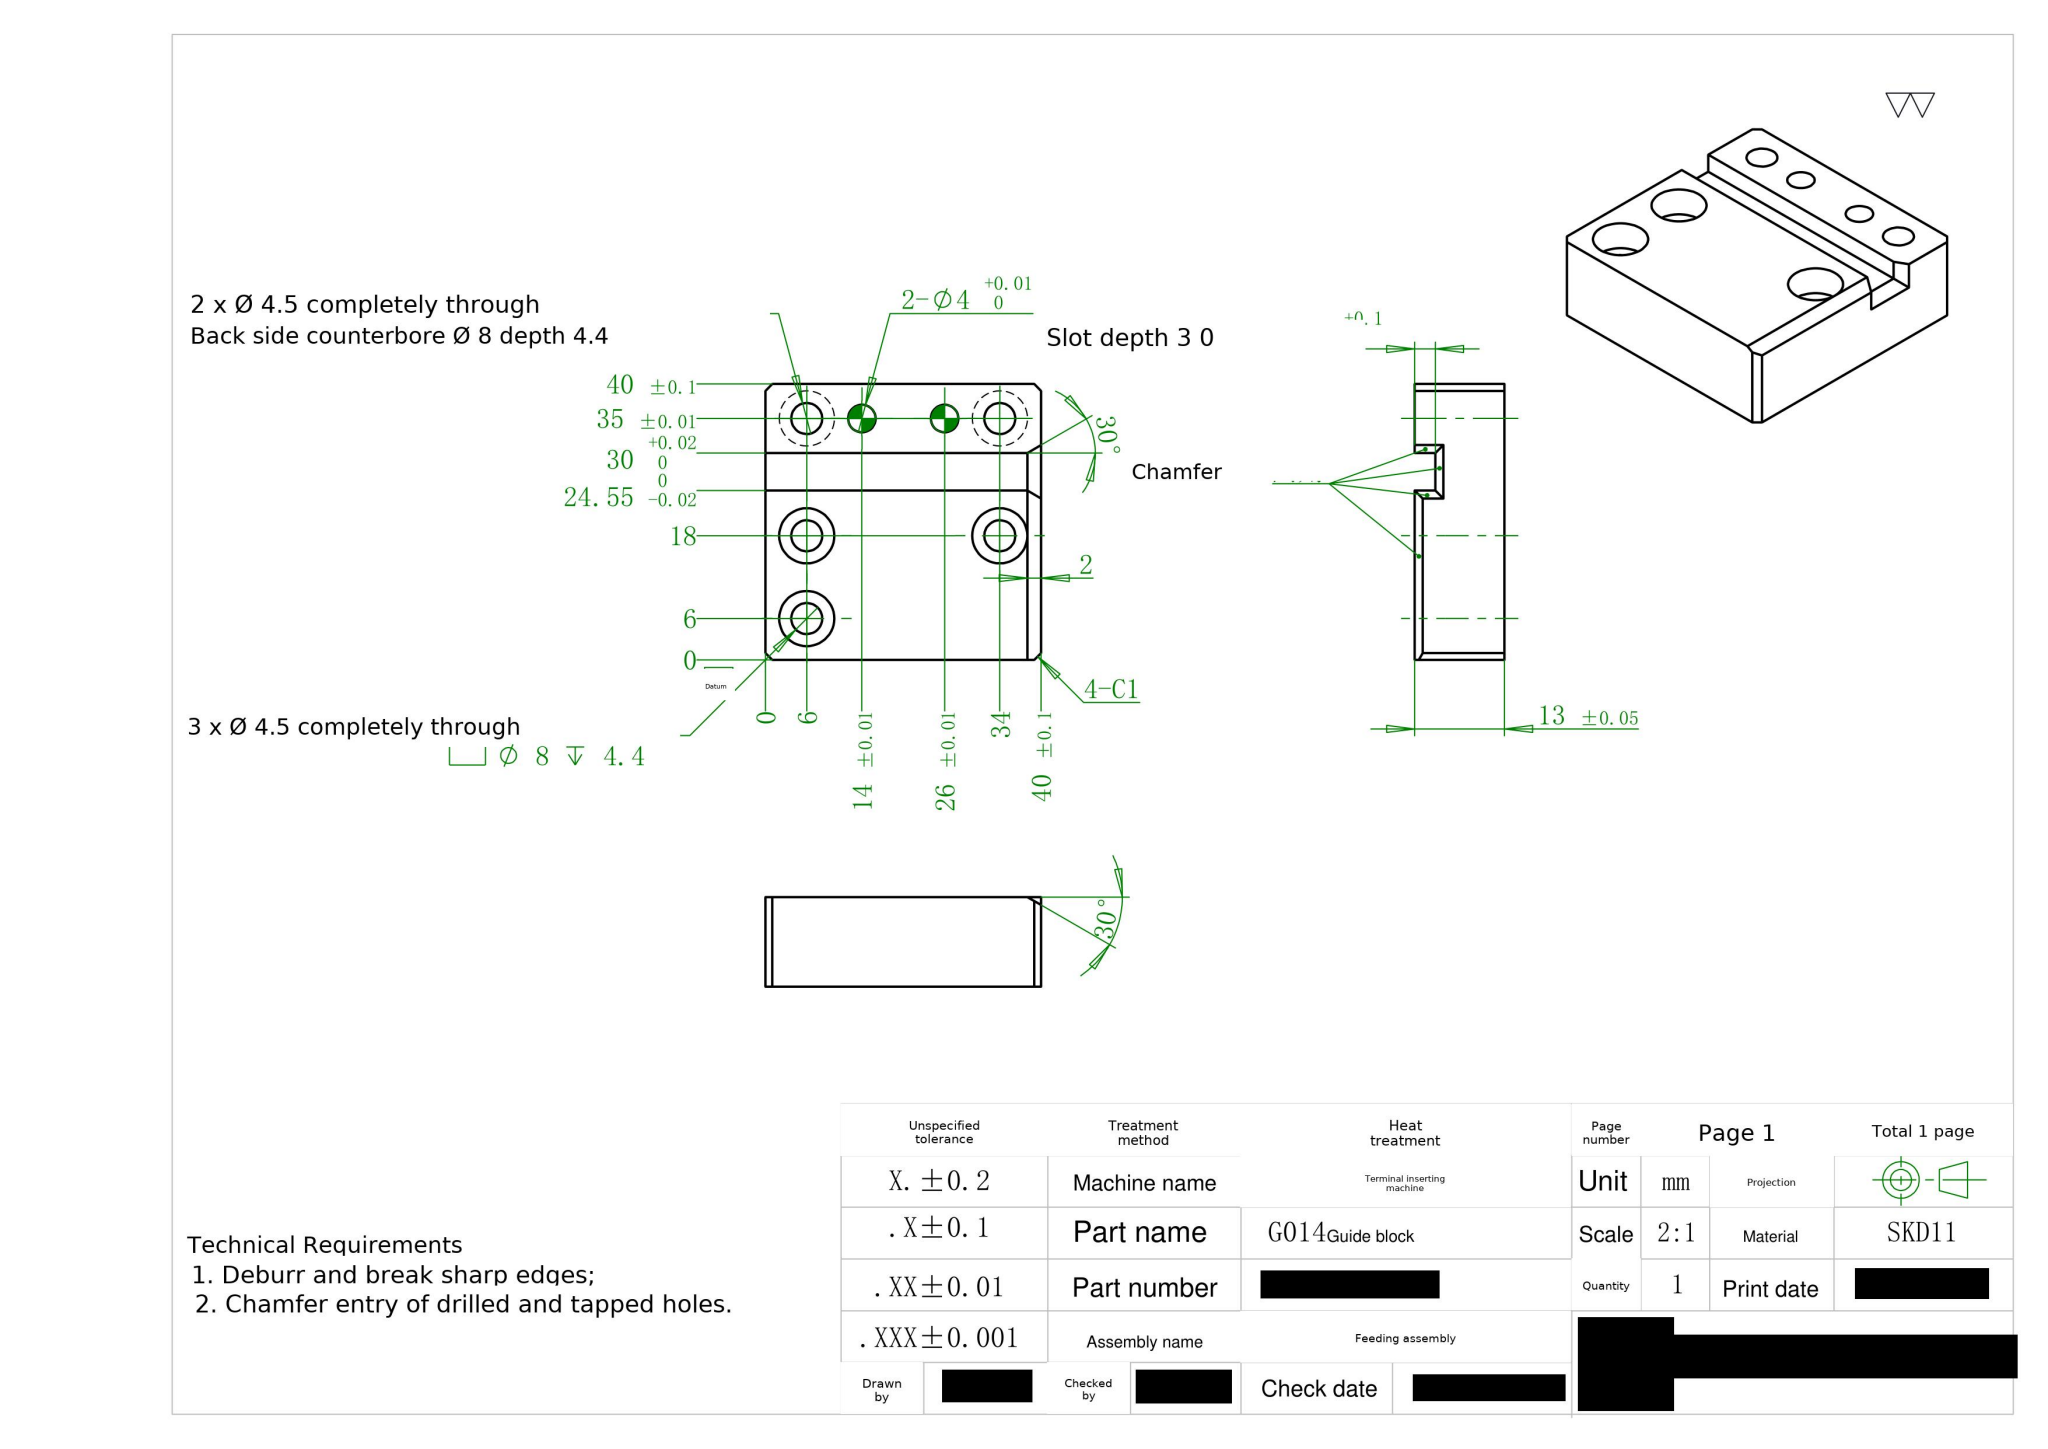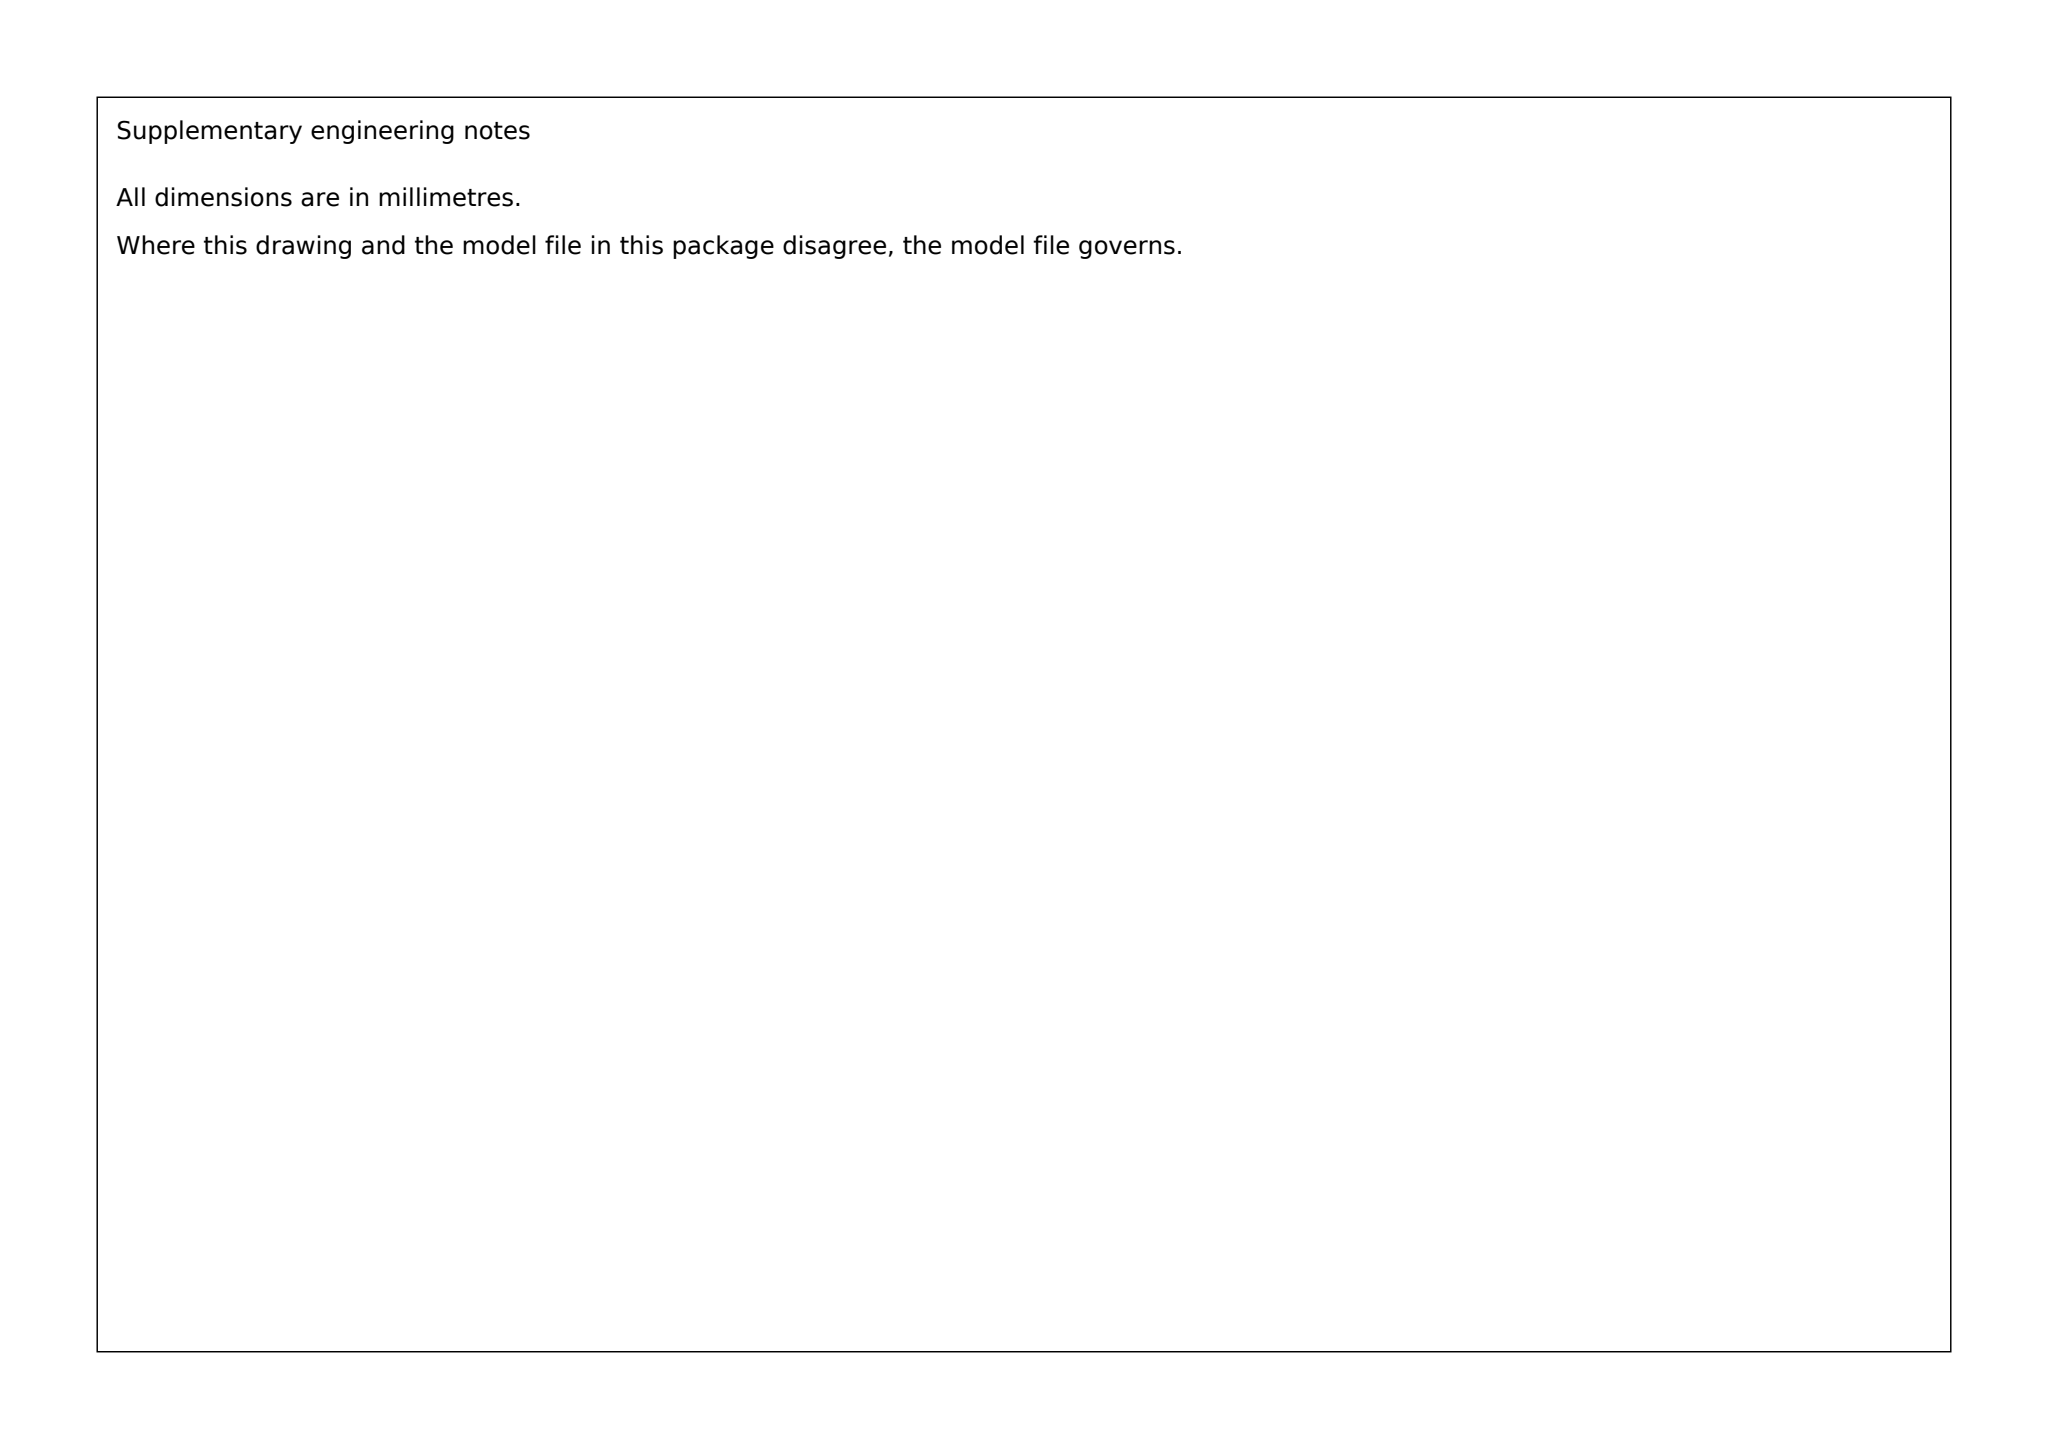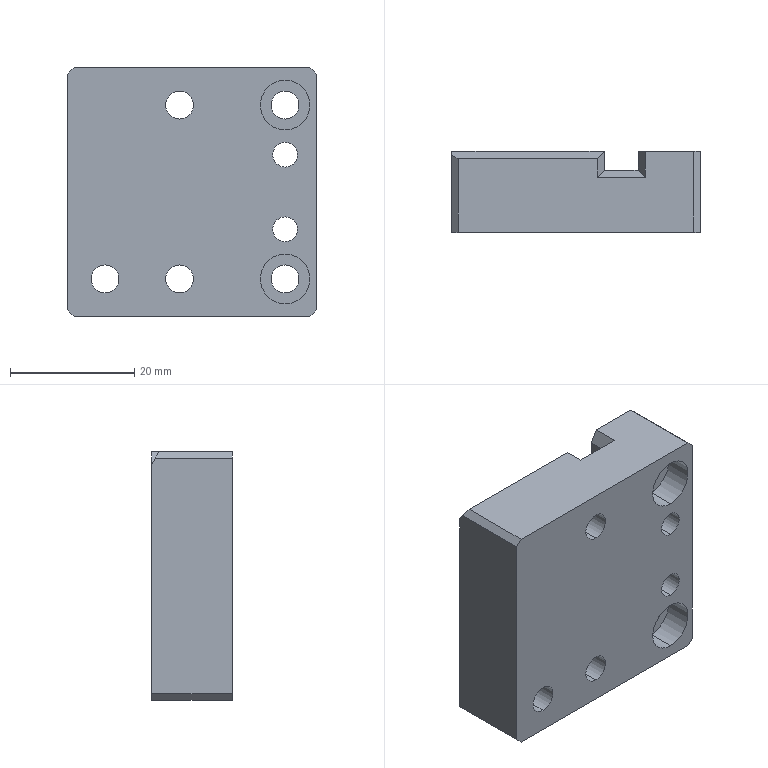Part | SolidWorks | mm | material SKD11 | 1 solid | 47 faces | box 40 x 13 x 40 mm | volume 17962 mm3 | cylinder 24 | plane 23 | commonest cylinder face diameters 8 x10 4.5 x10 4 x4